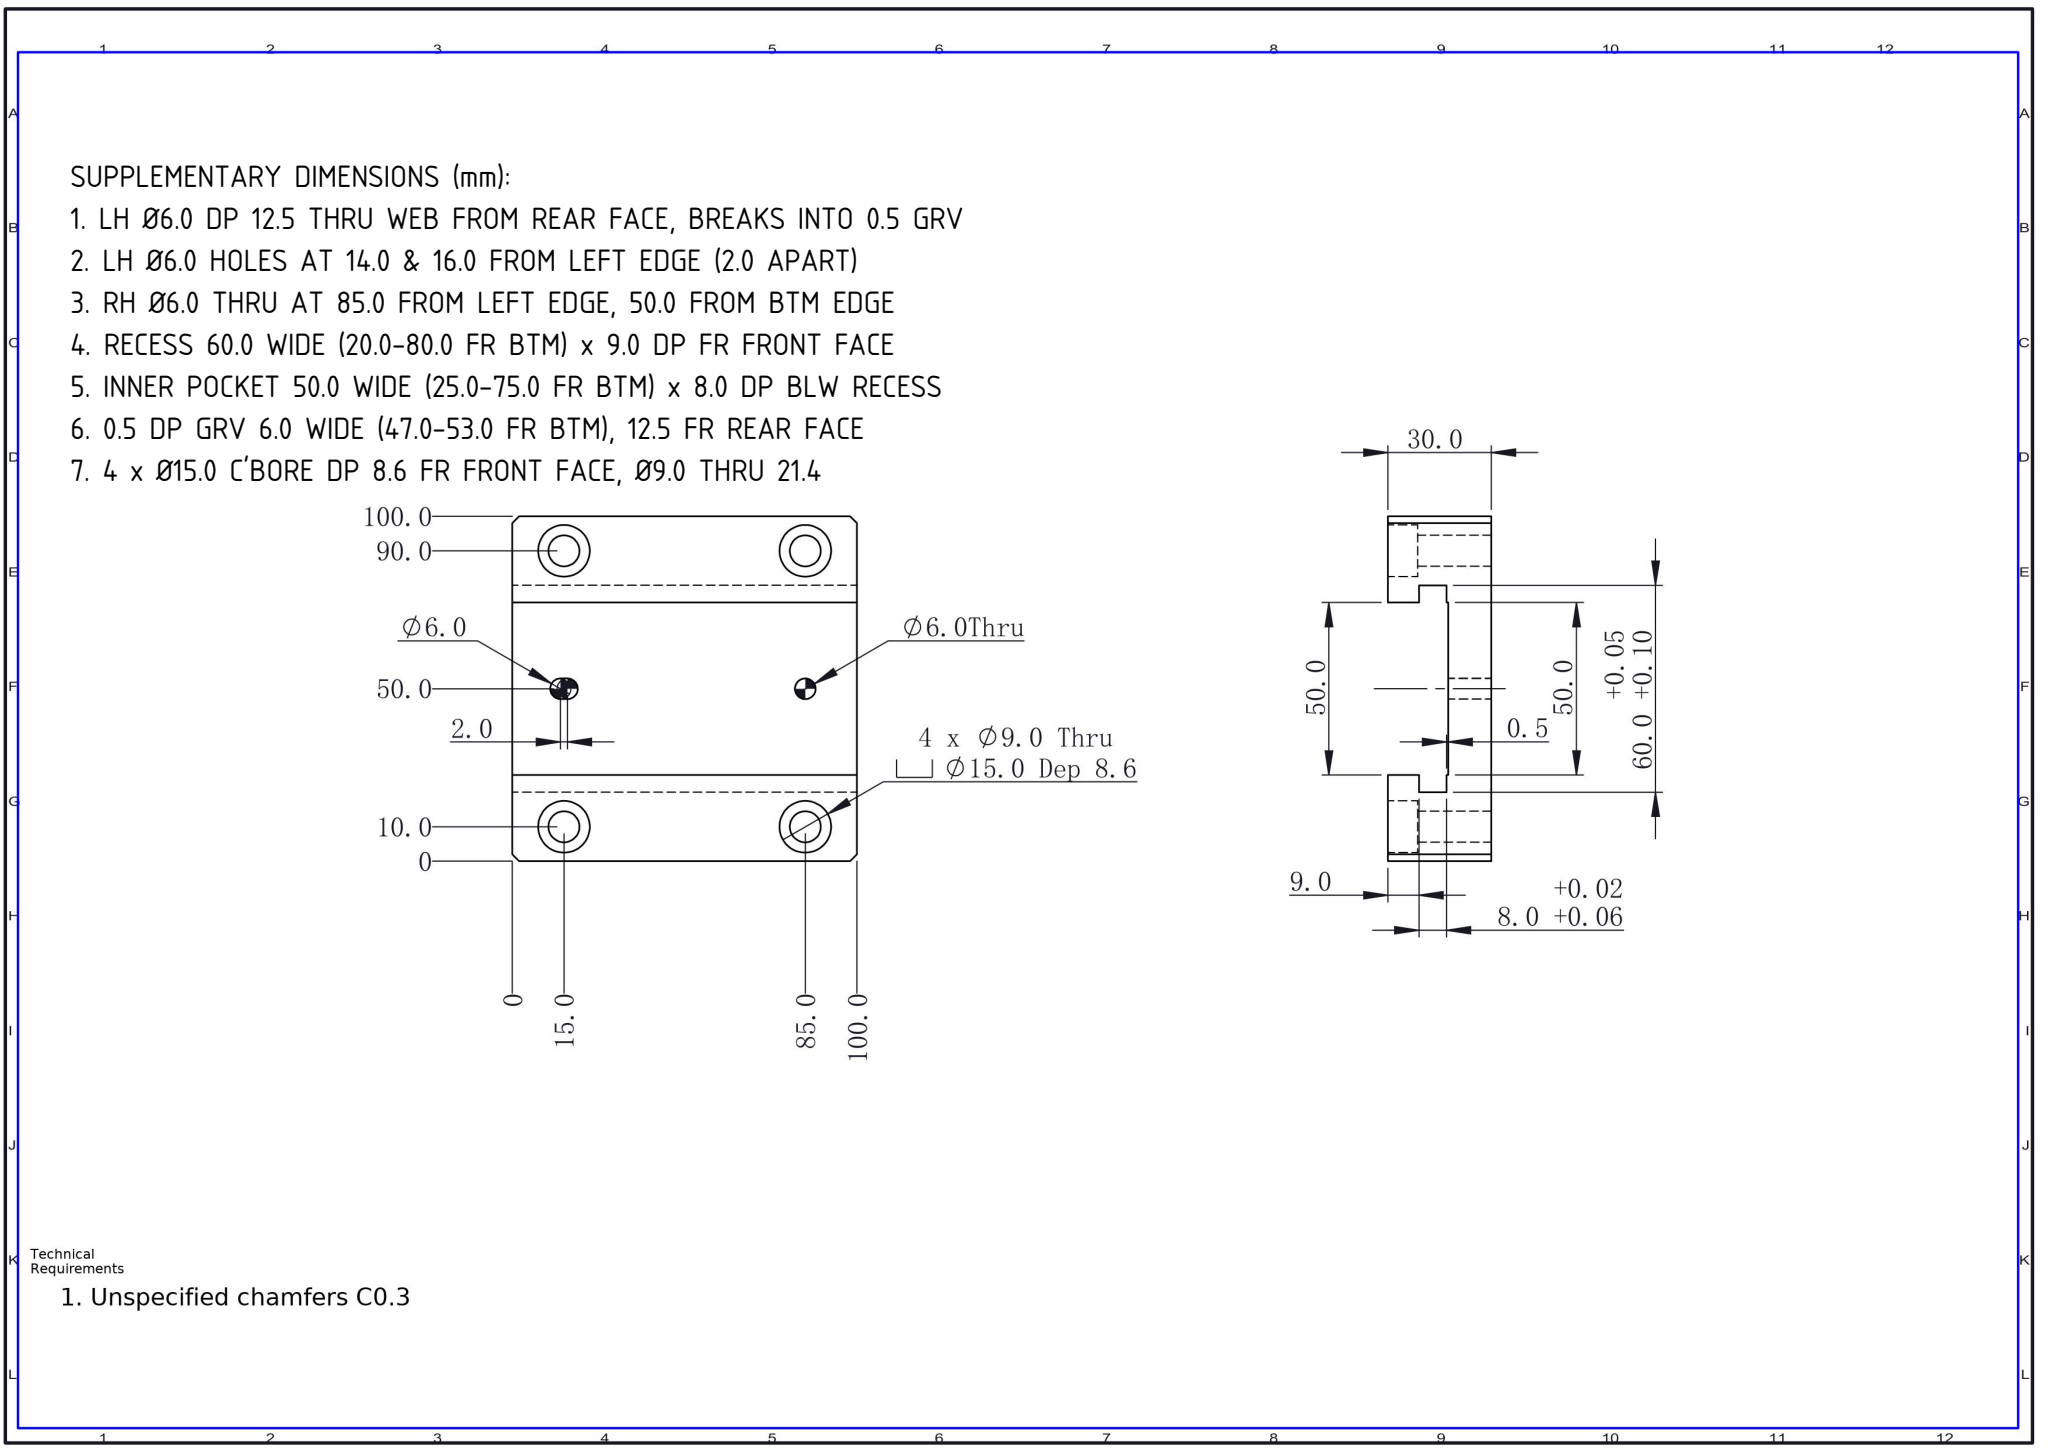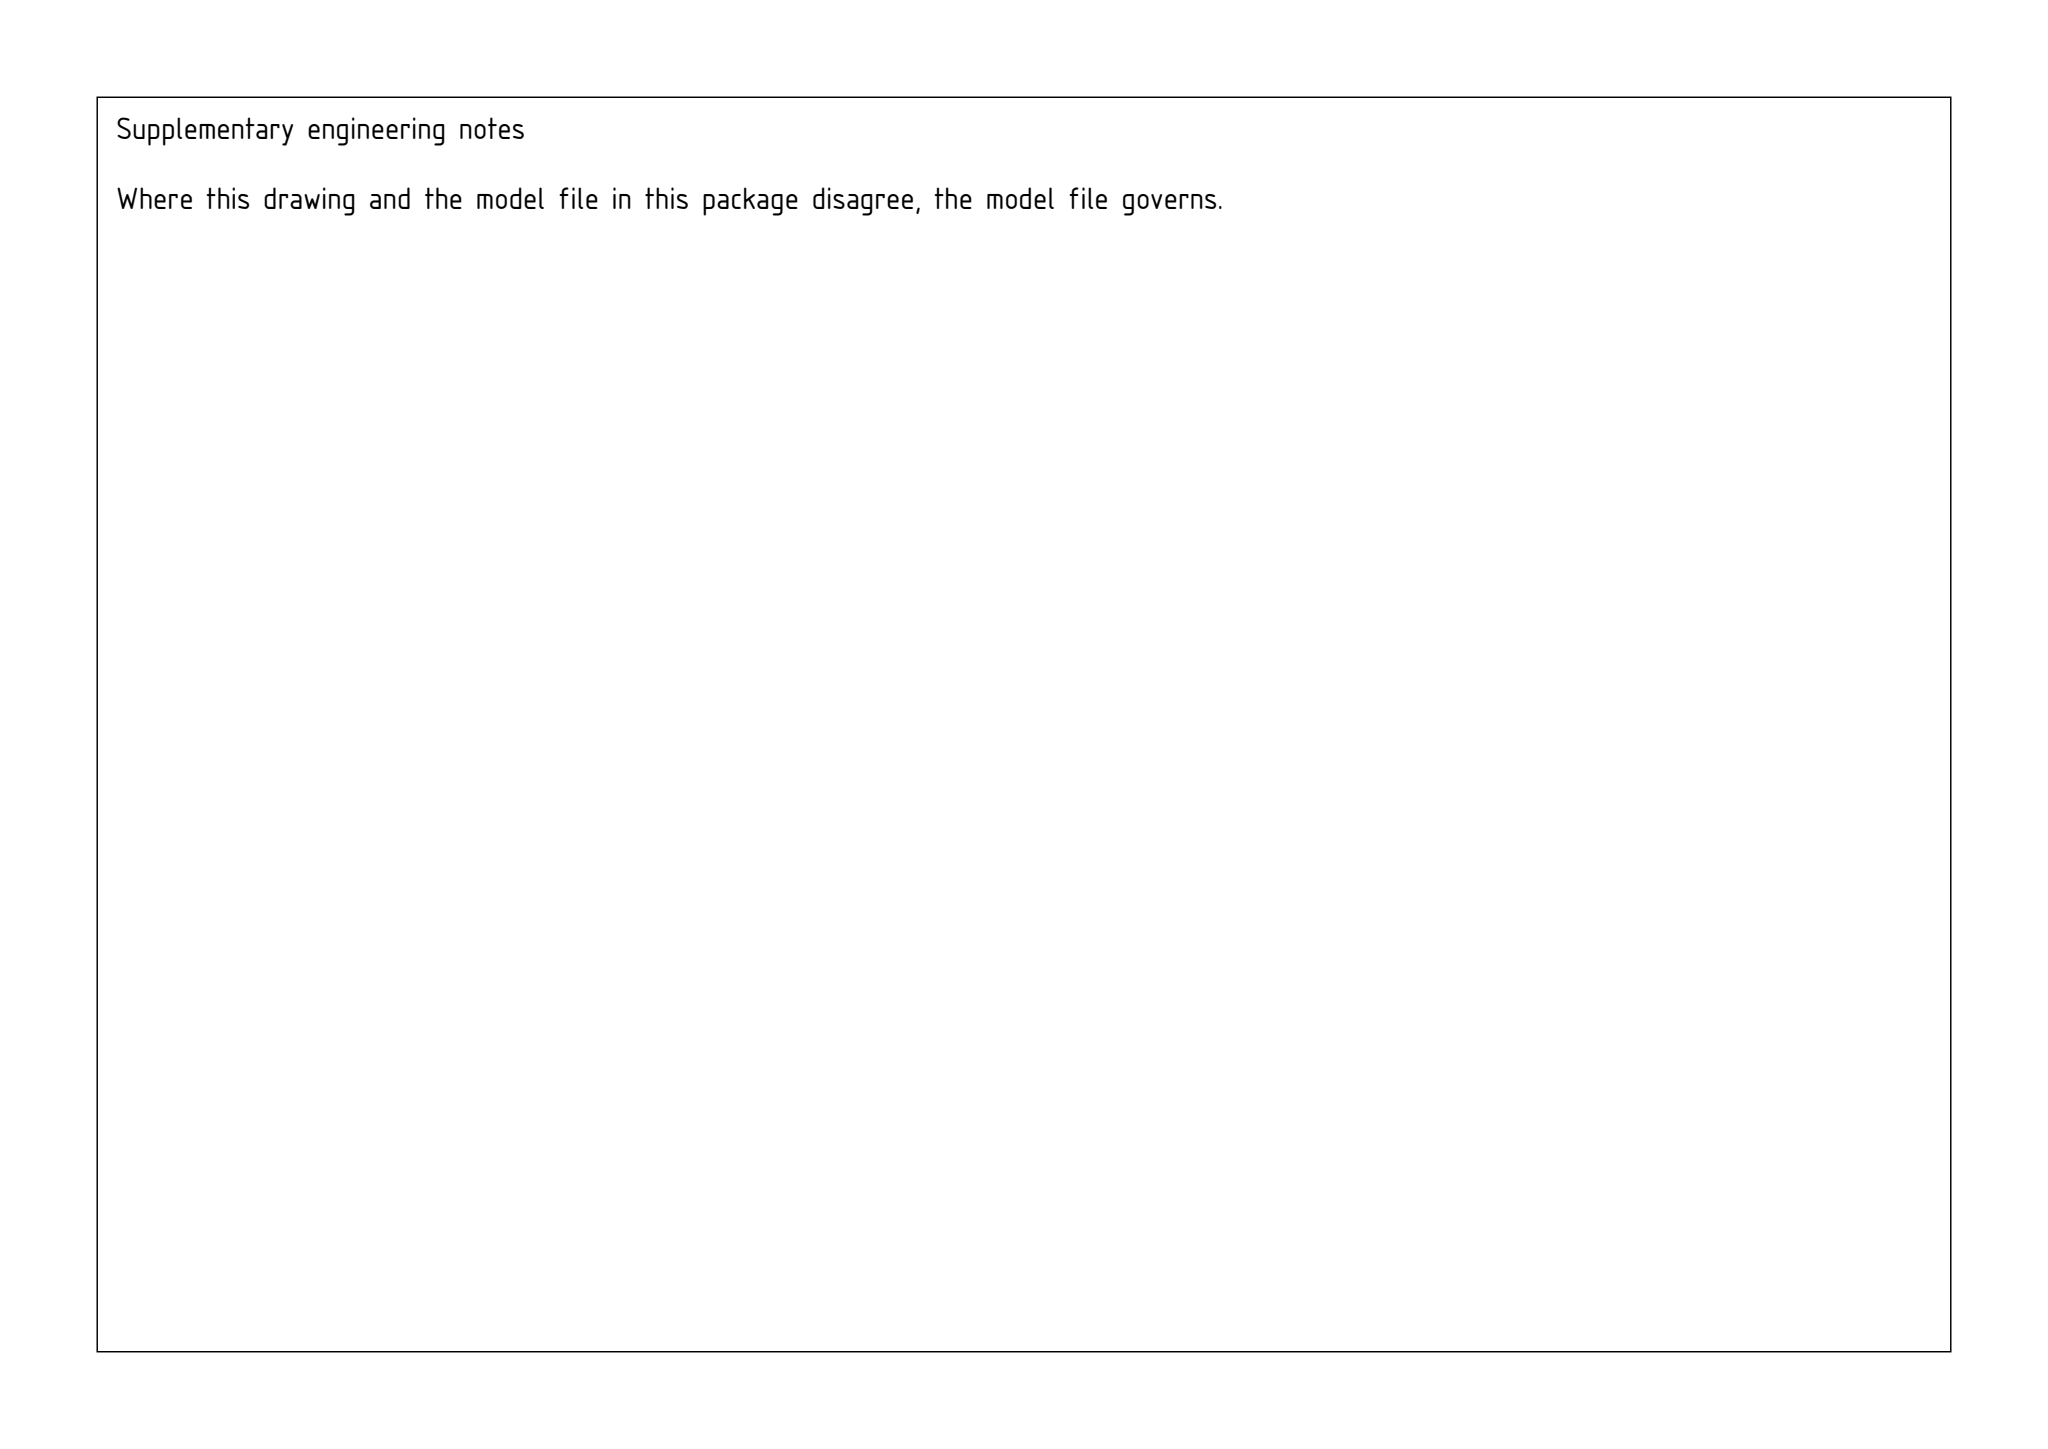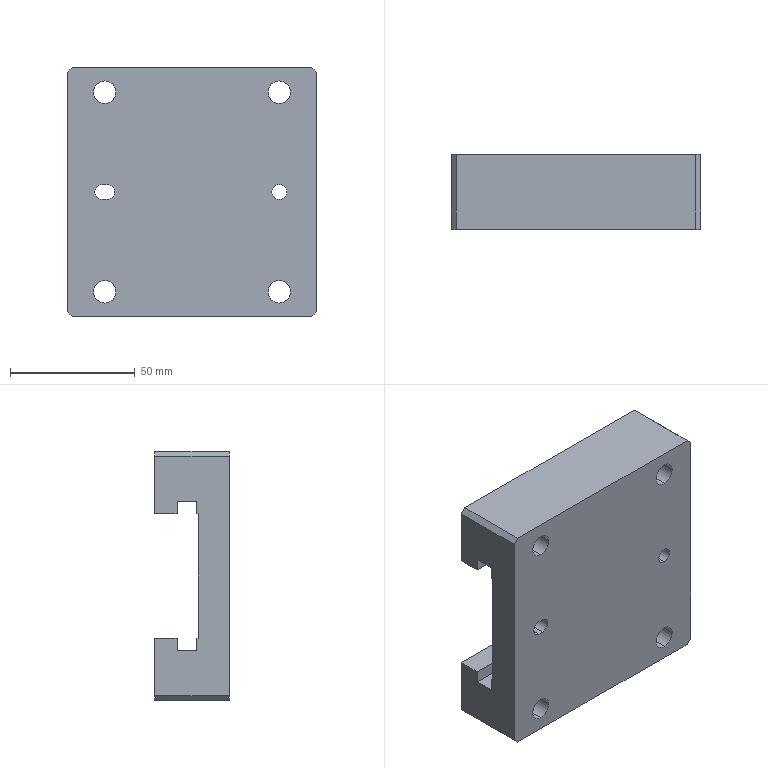Part | SolidWorks | mm | 1 solid | 48 faces | box 100 x 30 x 100 mm | volume 191879 mm3 | plane 28 | cylinder 20 | commonest cylinder face diameters 15 x8 9 x8 6 x4